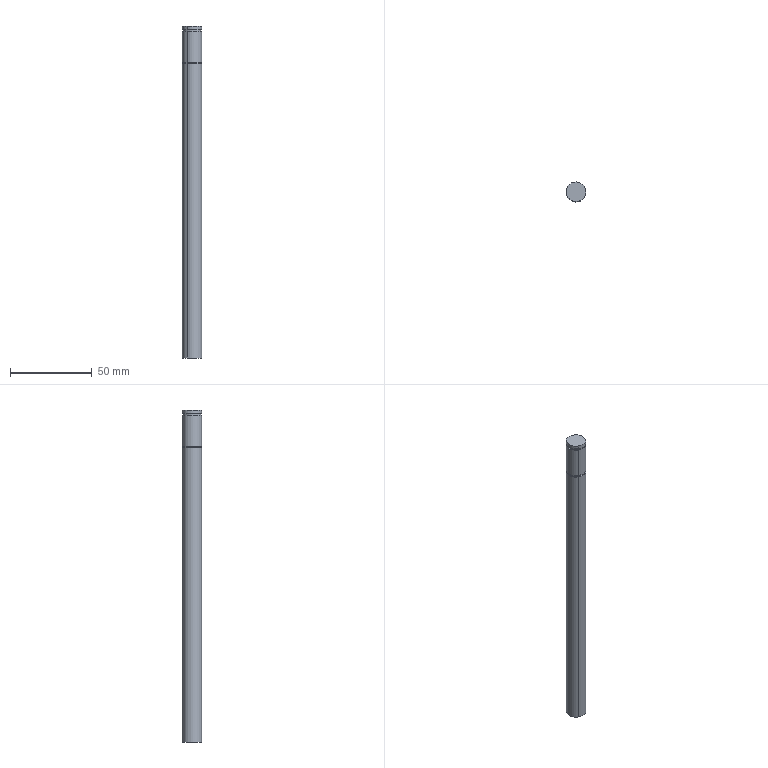Component | SolidWorks | TAR-02-026SmallPulleyAxis-1 | 1 solid | 16 faces | box 12 x 12 x 203 mm | volume 22911 mm3 | cylinder 10 | plane 6 | commonest cylinder face diameters 12 x6 10.8 x4
build123d program:
from build123d import *

# Parameters (mm, degrees)
SKETCH1_R           = 6
BOSS_EXTRUDE1_DEPTH = 2
SKETCH2_R           = 5.4
BOSS_EXTRUDE2_DEPTH = 1.1
SKETCH3_R           = 6
BOSS_EXTRUDE3_DEPTH = 19
SKETCH4_R           = 5.4
BOSS_EXTRUDE4_DEPTH = 1.1
SKETCH5_R           = 6
BOSS_EXTRUDE5_DEPTH = 179.8


with BuildPart() as part:
    # Sketch1 → Boss-Extrude1 (new body)
    with BuildSketch(Plane.XY):
        Circle(SKETCH1_R)
    extrude(amount=BOSS_EXTRUDE1_DEPTH)

    # Sketch2 → Boss-Extrude2 (add)
    with BuildSketch(Plane.XY.offset(2)):
        Circle(SKETCH2_R)
    extrude(amount=BOSS_EXTRUDE2_DEPTH)

    # Sketch3 → Boss-Extrude3 (add)
    with BuildSketch(Plane.XY.offset(3.1)):
        Circle(SKETCH3_R)
    extrude(amount=BOSS_EXTRUDE3_DEPTH)

    # Sketch4 → Boss-Extrude4 (add)
    with BuildSketch(Plane.XY.offset(22.1)):
        Circle(SKETCH4_R)
    extrude(amount=BOSS_EXTRUDE4_DEPTH)

    # Sketch5 → Boss-Extrude5 (add)
    with BuildSketch(Plane.XY.offset(23.2)):
        Circle(SKETCH5_R)
    extrude(amount=BOSS_EXTRUDE5_DEPTH)


solid = part.part

# Placed as in the assembly
solid = solid.moved(Location((-115.391, 9.288, 12.6), (180, 0, 0)))
STEP:
#1=COLOUR_RGB('',0.7922,0.8196,0.9333);
#2=FILL_AREA_STYLE_COLOUR('',#1);
#3=FILL_AREA_STYLE('',(#2));
#4=SURFACE_STYLE_FILL_AREA(#3);
#5=SURFACE_SIDE_STYLE('',(#4));
#6=SURFACE_STYLE_USAGE(.BOTH.,#5);
#7=PRESENTATION_STYLE_ASSIGNMENT((#6));
#8=CARTESIAN_POINT('',(-4.431,0.5734,-7.496));
#9=VERTEX_POINT('',#8);
#10=CARTESIAN_POINT('',(-4.655,0.1579,-7.496));
#11=VERTEX_POINT('',#10);
#12=CARTESIAN_POINT('',(-4.543,0.3657,-7.496));
#13=DIRECTION('',(0.,0.,-1.));
#14=DIRECTION('',(0.4758,0.8795,0.));
#15=AXIS2_PLACEMENT_3D('',#12,#13,#14);
#16=CIRCLE('',#15,0.2362);
#17=EDGE_CURVE('',#9,#11,#16,.T.);
#18=ORIENTED_EDGE('',*,*,#17,.F.);
#19=CARTESIAN_POINT('',(-4.431,0.5734,-0.4173));
#20=VERTEX_POINT('',#19);
#21=CARTESIAN_POINT('',(-4.431,0.5734,-7.496));
#22=DIRECTION('',(0.,0.,1.));
#23=VECTOR('',#22,39.37);
#24=LINE('',#21,#23);
#25=EDGE_CURVE('',#9,#20,#24,.T.);
#26=ORIENTED_EDGE('',*,*,#25,.T.);
#27=CARTESIAN_POINT('',(-4.655,0.1579,-0.4173));
#28=VERTEX_POINT('',#27);
#29=CARTESIAN_POINT('',(-4.543,0.3657,-0.4173));
#30=DIRECTION('',(0.,0.,-1.));
#31=DIRECTION('',(0.4758,0.8795,0.));
#32=AXIS2_PLACEMENT_3D('',#29,#30,#31);
#33=CIRCLE('',#32,0.2362);
#34=EDGE_CURVE('',#20,#28,#33,.T.);
#35=ORIENTED_EDGE('',*,*,#34,.T.);
#36=CARTESIAN_POINT('',(-4.655,0.1579,-7.496));
#37=DIRECTION('',(0.,0.,1.));
#38=VECTOR('',#37,39.37);
#39=LINE('',#36,#38);
#40=EDGE_CURVE('',#11,#28,#39,.T.);
#41=ORIENTED_EDGE('',*,*,#40,.F.);
#42=EDGE_LOOP('',(#18,#26,#35,#41));
#43=FACE_OUTER_BOUND('',#42,.T.);
#44=CARTESIAN_POINT('',(-4.543,0.3657,-7.496));
#45=DIRECTION('',(0.,0.,1.));
#46=DIRECTION('',(-0.4758,-0.8795,0.));
#47=AXIS2_PLACEMENT_3D('',#44,#45,#46);
#48=CYLINDRICAL_SURFACE('',#47,0.2362);
#49=ADVANCED_FACE('',(#43),#48,.T.);
#50=CARTESIAN_POINT('',(-4.442,0.5526,-0.4173));
#51=VERTEX_POINT('',#50);
#52=CARTESIAN_POINT('',(-4.644,0.1787,-0.4173));
#53=VERTEX_POINT('',#52);
#54=CARTESIAN_POINT('',(-4.543,0.3657,-0.4173));
#55=DIRECTION('',(0.,0.,-1.));
#56=DIRECTION('',(0.4758,0.8795,0.));
#57=AXIS2_PLACEMENT_3D('',#54,#55,#56);
#58=CIRCLE('',#57,0.2126);
#59=EDGE_CURVE('',#51,#53,#58,.T.);
#60=ORIENTED_EDGE('',*,*,#59,.F.);
#61=CARTESIAN_POINT('',(-4.442,0.5526,-0.374));
#62=VERTEX_POINT('',#61);
#63=CARTESIAN_POINT('',(-4.442,0.5526,-0.4173));
#64=DIRECTION('',(0.,0.,1.));
#65=VECTOR('',#64,39.37);
#66=LINE('',#63,#65);
#67=EDGE_CURVE('',#51,#62,#66,.T.);
#68=ORIENTED_EDGE('',*,*,#67,.T.);
#69=CARTESIAN_POINT('',(-4.644,0.1787,-0.374));
#70=VERTEX_POINT('',#69);
#71=CARTESIAN_POINT('',(-4.543,0.3657,-0.374));
#72=DIRECTION('',(0.,0.,-1.));
#73=DIRECTION('',(0.4758,0.8795,0.));
#74=AXIS2_PLACEMENT_3D('',#71,#72,#73);
#75=CIRCLE('',#74,0.2126);
#76=EDGE_CURVE('',#62,#70,#75,.T.);
#77=ORIENTED_EDGE('',*,*,#76,.T.);
#78=CARTESIAN_POINT('',(-4.644,0.1787,-0.4173));
#79=DIRECTION('',(0.,0.,1.));
#80=VECTOR('',#79,39.37);
#81=LINE('',#78,#80);
#82=EDGE_CURVE('',#53,#70,#81,.T.);
#83=ORIENTED_EDGE('',*,*,#82,.F.);
#84=EDGE_LOOP('',(#60,#68,#77,#83));
#85=FACE_OUTER_BOUND('',#84,.T.);
#86=CARTESIAN_POINT('',(-4.543,0.3657,-0.4173));
#87=DIRECTION('',(0.,0.,1.));
#88=DIRECTION('',(-0.4758,-0.8795,0.));
#89=AXIS2_PLACEMENT_3D('',#86,#87,#88);
#90=CYLINDRICAL_SURFACE('',#89,0.2126);
#91=ADVANCED_FACE('',(#85),#90,.T.);
#92=CARTESIAN_POINT('',(-4.431,0.5734,-0.374));
#93=VERTEX_POINT('',#92);
#94=CARTESIAN_POINT('',(-4.655,0.1579,-0.374));
#95=VERTEX_POINT('',#94);
#96=CARTESIAN_POINT('',(-4.543,0.3657,-0.374));
#97=DIRECTION('',(0.,0.,-1.));
#98=DIRECTION('',(0.4758,0.8795,0.));
#99=AXIS2_PLACEMENT_3D('',#96,#97,#98);
#100=CIRCLE('',#99,0.2362);
#101=EDGE_CURVE('',#93,#95,#100,.T.);
#102=ORIENTED_EDGE('',*,*,#101,.F.);
#103=CARTESIAN_POINT('',(-4.431,0.5734,0.374));
#104=VERTEX_POINT('',#103);
#105=CARTESIAN_POINT('',(-4.431,0.5734,-0.374));
#106=DIRECTION('',(0.,0.,1.));
#107=VECTOR('',#106,39.37);
#108=LINE('',#105,#107);
#109=EDGE_CURVE('',#93,#104,#108,.T.);
#110=ORIENTED_EDGE('',*,*,#109,.T.);
#111=CARTESIAN_POINT('',(-4.655,0.1579,0.374));
#112=VERTEX_POINT('',#111);
#113=CARTESIAN_POINT('',(-4.543,0.3657,0.374));
#114=DIRECTION('',(0.,0.,-1.));
#115=DIRECTION('',(0.4758,0.8795,0.));
#116=AXIS2_PLACEMENT_3D('',#113,#114,#115);
#117=CIRCLE('',#116,0.2362);
#118=EDGE_CURVE('',#104,#112,#117,.T.);
#119=ORIENTED_EDGE('',*,*,#118,.T.);
#120=CARTESIAN_POINT('',(-4.655,0.1579,-0.374));
#121=DIRECTION('',(0.,0.,1.));
#122=VECTOR('',#121,39.37);
#123=LINE('',#120,#122);
#124=EDGE_CURVE('',#95,#112,#123,.T.);
#125=ORIENTED_EDGE('',*,*,#124,.F.);
#126=EDGE_LOOP('',(#102,#110,#119,#125));
#127=FACE_OUTER_BOUND('',#126,.T.);
#128=CARTESIAN_POINT('',(-4.543,0.3657,-0.374));
#129=DIRECTION('',(0.,0.,1.));
#130=DIRECTION('',(-0.4758,-0.8795,0.));
#131=AXIS2_PLACEMENT_3D('',#128,#129,#130);
#132=CYLINDRICAL_SURFACE('',#131,0.2362);
#133=ADVANCED_FACE('',(#127),#132,.T.);
#134=CARTESIAN_POINT('',(-4.442,0.5526,0.374));
#135=VERTEX_POINT('',#134);
#136=CARTESIAN_POINT('',(-4.644,0.1787,0.374));
#137=VERTEX_POINT('',#136);
#138=CARTESIAN_POINT('',(-4.543,0.3657,0.374));
#139=DIRECTION('',(0.,0.,-1.));
#140=DIRECTION('',(0.4758,0.8795,0.));
#141=AXIS2_PLACEMENT_3D('',#138,#139,#140);
#142=CIRCLE('',#141,0.2126);
#143=EDGE_CURVE('',#135,#137,#142,.T.);
#144=ORIENTED_EDGE('',*,*,#143,.F.);
#145=CARTESIAN_POINT('',(-4.442,0.5526,0.4173));
#146=VERTEX_POINT('',#145);
#147=CARTESIAN_POINT('',(-4.442,0.5526,0.374));
#148=DIRECTION('',(0.,0.,1.));
#149=VECTOR('',#148,39.37);
#150=LINE('',#147,#149);
#151=EDGE_CURVE('',#135,#146,#150,.T.);
#152=ORIENTED_EDGE('',*,*,#151,.T.);
#153=CARTESIAN_POINT('',(-4.644,0.1787,0.4173));
#154=VERTEX_POINT('',#153);
#155=CARTESIAN_POINT('',(-4.543,0.3657,0.4173));
#156=DIRECTION('',(0.,0.,-1.));
#157=DIRECTION('',(0.4758,0.8795,0.));
#158=AXIS2_PLACEMENT_3D('',#155,#156,#157);
#159=CIRCLE('',#158,0.2126);
#160=EDGE_CURVE('',#146,#154,#159,.T.);
#161=ORIENTED_EDGE('',*,*,#160,.T.);
#162=CARTESIAN_POINT('',(-4.644,0.1787,0.374));
#163=DIRECTION('',(0.,0.,1.));
#164=VECTOR('',#163,39.37);
#165=LINE('',#162,#164);
#166=EDGE_CURVE('',#137,#154,#165,.T.);
#167=ORIENTED_EDGE('',*,*,#166,.F.);
#168=EDGE_LOOP('',(#144,#152,#161,#167));
#169=FACE_OUTER_BOUND('',#168,.T.);
#170=CARTESIAN_POINT('',(-4.543,0.3657,0.374));
#171=DIRECTION('',(0.,0.,1.));
#172=DIRECTION('',(-0.4758,-0.8795,0.));
#173=AXIS2_PLACEMENT_3D('',#170,#171,#172);
#174=CYLINDRICAL_SURFACE('',#173,0.2126);
#175=ADVANCED_FACE('',(#169),#174,.T.);
#176=CARTESIAN_POINT('',(-4.431,0.5734,0.4173));
#177=VERTEX_POINT('',#176);
#178=CARTESIAN_POINT('',(-4.655,0.1579,0.4173));
#179=VERTEX_POINT('',#178);
#180=CARTESIAN_POINT('',(-4.543,0.3657,0.4173));
#181=DIRECTION('',(0.,0.,-1.));
#182=DIRECTION('',(0.4758,0.8795,0.));
#183=AXIS2_PLACEMENT_3D('',#180,#181,#182);
#184=CIRCLE('',#183,0.2362);
#185=EDGE_CURVE('',#177,#179,#184,.T.);
#186=ORIENTED_EDGE('',*,*,#185,.F.);
#187=CARTESIAN_POINT('',(-4.431,0.5734,0.4961));
#188=VERTEX_POINT('',#187);
#189=CARTESIAN_POINT('',(-4.431,0.5734,0.4173));
#190=DIRECTION('',(0.,0.,1.));
#191=VECTOR('',#190,39.37);
#192=LINE('',#189,#191);
#193=EDGE_CURVE('',#177,#188,#192,.T.);
#194=ORIENTED_EDGE('',*,*,#193,.T.);
#195=CARTESIAN_POINT('',(-4.655,0.1579,0.4961));
#196=VERTEX_POINT('',#195);
#197=CARTESIAN_POINT('',(-4.543,0.3657,0.4961));
#198=DIRECTION('',(0.,0.,-1.));
#199=DIRECTION('',(0.4758,0.8795,0.));
#200=AXIS2_PLACEMENT_3D('',#197,#198,#199);
#201=CIRCLE('',#200,0.2362);
#202=EDGE_CURVE('',#188,#196,#201,.T.);
#203=ORIENTED_EDGE('',*,*,#202,.T.);
#204=CARTESIAN_POINT('',(-4.655,0.1579,0.4173));
#205=DIRECTION('',(0.,0.,1.));
#206=VECTOR('',#205,39.37);
#207=LINE('',#204,#206);
#208=EDGE_CURVE('',#179,#196,#207,.T.);
#209=ORIENTED_EDGE('',*,*,#208,.F.);
#210=EDGE_LOOP('',(#186,#194,#203,#209));
#211=FACE_OUTER_BOUND('',#210,.T.);
#212=CARTESIAN_POINT('',(-4.543,0.3657,0.4173));
#213=DIRECTION('',(0.,0.,1.));
#214=DIRECTION('',(-0.4758,-0.8795,0.));
#215=AXIS2_PLACEMENT_3D('',#212,#213,#214);
#216=CYLINDRICAL_SURFACE('',#215,0.2362);
#217=ADVANCED_FACE('',(#211),#216,.T.);
#218=ORIENTED_EDGE('',*,*,#193,.F.);
#219=CARTESIAN_POINT('',(-4.543,0.3657,0.4173));
#220=DIRECTION('',(0.,0.,-1.));
#221=DIRECTION('',(0.4758,0.8795,0.));
#222=AXIS2_PLACEMENT_3D('',#219,#220,#221);
#223=CIRCLE('',#222,0.2362);
#224=EDGE_CURVE('',#179,#177,#223,.T.);
#225=ORIENTED_EDGE('',*,*,#224,.F.);
#226=ORIENTED_EDGE('',*,*,#208,.T.);
#227=CARTESIAN_POINT('',(-4.543,0.3657,0.4961));
#228=DIRECTION('',(0.,0.,-1.));
#229=DIRECTION('',(0.4758,0.8795,0.));
#230=AXIS2_PLACEMENT_3D('',#227,#228,#229);
#231=CIRCLE('',#230,0.2362);
#232=EDGE_CURVE('',#196,#188,#231,.T.);
#233=ORIENTED_EDGE('',*,*,#232,.T.);
#234=EDGE_LOOP('',(#218,#225,#226,#233));
#235=FACE_OUTER_BOUND('',#234,.T.);
#236=CARTESIAN_POINT('',(-4.543,0.3657,0.4173));
#237=DIRECTION('',(0.,0.,1.));
#238=DIRECTION('',(-0.4758,-0.8795,0.));
#239=AXIS2_PLACEMENT_3D('',#236,#237,#238);
#240=CYLINDRICAL_SURFACE('',#239,0.2362);
#241=ADVANCED_FACE('',(#235),#240,.T.);
#242=CARTESIAN_POINT('',(-4.543,0.3657,0.4173));
#243=DIRECTION('',(0.,0.,-1.));
#244=DIRECTION('',(0.4758,0.8795,0.));
#245=AXIS2_PLACEMENT_3D('',#242,#243,#244);
#246=CIRCLE('',#245,0.2126);
#247=EDGE_CURVE('',#154,#146,#246,.T.);
#248=ORIENTED_EDGE('',*,*,#247,.F.);
#249=ORIENTED_EDGE('',*,*,#160,.F.);
#250=EDGE_LOOP('',(#248,#249));
#251=FACE_BOUND('',#250,.T.);
#252=ORIENTED_EDGE('',*,*,#224,.T.);
#253=ORIENTED_EDGE('',*,*,#185,.T.);
#254=EDGE_LOOP('',(#252,#253));
#255=FACE_OUTER_BOUND('',#254,.T.);
#256=CARTESIAN_POINT('',(-4.543,0.3657,0.4173));
#257=DIRECTION('',(0.,0.,-1.));
#258=DIRECTION('',(0.4758,0.8795,0.));
#259=AXIS2_PLACEMENT_3D('',#256,#257,#258);
#260=PLANE('',#259);
#261=ADVANCED_FACE('',(#251,#255),#260,.T.);
#262=ORIENTED_EDGE('',*,*,#232,.F.);
#263=ORIENTED_EDGE('',*,*,#202,.F.);
#264=EDGE_LOOP('',(#262,#263));
#265=FACE_OUTER_BOUND('',#264,.T.);
#266=CARTESIAN_POINT('',(-4.543,0.3657,0.4961));
#267=DIRECTION('',(0.,0.,-1.));
#268=DIRECTION('',(0.4758,0.8795,0.));
#269=AXIS2_PLACEMENT_3D('',#266,#267,#268);
#270=PLANE('',#269);
#271=ADVANCED_FACE('',(#265),#270,.F.);
#272=ORIENTED_EDGE('',*,*,#151,.F.);
#273=CARTESIAN_POINT('',(-4.543,0.3657,0.374));
#274=DIRECTION('',(0.,0.,-1.));
#275=DIRECTION('',(0.4758,0.8795,0.));
#276=AXIS2_PLACEMENT_3D('',#273,#274,#275);
#277=CIRCLE('',#276,0.2126);
#278=EDGE_CURVE('',#137,#135,#277,.T.);
#279=ORIENTED_EDGE('',*,*,#278,.F.);
#280=ORIENTED_EDGE('',*,*,#166,.T.);
#281=ORIENTED_EDGE('',*,*,#247,.T.);
#282=EDGE_LOOP('',(#272,#279,#280,#281));
#283=FACE_OUTER_BOUND('',#282,.T.);
#284=CARTESIAN_POINT('',(-4.543,0.3657,0.374));
#285=DIRECTION('',(0.,0.,1.));
#286=DIRECTION('',(-0.4758,-0.8795,0.));
#287=AXIS2_PLACEMENT_3D('',#284,#285,#286);
#288=CYLINDRICAL_SURFACE('',#287,0.2126);
#289=ADVANCED_FACE('',(#283),#288,.T.);
#290=ORIENTED_EDGE('',*,*,#109,.F.);
#291=CARTESIAN_POINT('',(-4.543,0.3657,-0.374));
#292=DIRECTION('',(0.,0.,-1.));
#293=DIRECTION('',(0.4758,0.8795,0.));
#294=AXIS2_PLACEMENT_3D('',#291,#292,#293);
#295=CIRCLE('',#294,0.2362);
#296=EDGE_CURVE('',#95,#93,#295,.T.);
#297=ORIENTED_EDGE('',*,*,#296,.F.);
#298=ORIENTED_EDGE('',*,*,#124,.T.);
#299=CARTESIAN_POINT('',(-4.543,0.3657,0.374));
#300=DIRECTION('',(0.,0.,-1.));
#301=DIRECTION('',(0.4758,0.8795,0.));
#302=AXIS2_PLACEMENT_3D('',#299,#300,#301);
#303=CIRCLE('',#302,0.2362);
#304=EDGE_CURVE('',#112,#104,#303,.T.);
#305=ORIENTED_EDGE('',*,*,#304,.T.);
#306=EDGE_LOOP('',(#290,#297,#298,#305));
#307=FACE_OUTER_BOUND('',#306,.T.);
#308=CARTESIAN_POINT('',(-4.543,0.3657,-0.374));
#309=DIRECTION('',(0.,0.,1.));
#310=DIRECTION('',(-0.4758,-0.8795,0.));
#311=AXIS2_PLACEMENT_3D('',#308,#309,#310);
#312=CYLINDRICAL_SURFACE('',#311,0.2362);
#313=ADVANCED_FACE('',(#307),#312,.T.);
#314=CARTESIAN_POINT('',(-4.543,0.3657,-0.374));
#315=DIRECTION('',(0.,0.,-1.));
#316=DIRECTION('',(0.4758,0.8795,0.));
#317=AXIS2_PLACEMENT_3D('',#314,#315,#316);
#318=CIRCLE('',#317,0.2126);
#319=EDGE_CURVE('',#70,#62,#318,.T.);
#320=ORIENTED_EDGE('',*,*,#319,.F.);
#321=ORIENTED_EDGE('',*,*,#76,.F.);
#322=EDGE_LOOP('',(#320,#321));
#323=FACE_BOUND('',#322,.T.);
#324=ORIENTED_EDGE('',*,*,#296,.T.);
#325=ORIENTED_EDGE('',*,*,#101,.T.);
#326=EDGE_LOOP('',(#324,#325));
#327=FACE_OUTER_BOUND('',#326,.T.);
#328=CARTESIAN_POINT('',(-4.543,0.3657,-0.374));
#329=DIRECTION('',(0.,0.,-1.));
#330=DIRECTION('',(0.4758,0.8795,0.));
#331=AXIS2_PLACEMENT_3D('',#328,#329,#330);
#332=PLANE('',#331);
#333=ADVANCED_FACE('',(#323,#327),#332,.T.);
#334=ORIENTED_EDGE('',*,*,#278,.T.);
#335=ORIENTED_EDGE('',*,*,#143,.T.);
#336=EDGE_LOOP('',(#334,#335));
#337=FACE_BOUND('',#336,.T.);
#338=ORIENTED_EDGE('',*,*,#304,.F.);
#339=ORIENTED_EDGE('',*,*,#118,.F.);
#340=EDGE_LOOP('',(#338,#339));
#341=FACE_OUTER_BOUND('',#340,.T.);
#342=CARTESIAN_POINT('',(-4.543,0.3657,0.374));
#343=DIRECTION('',(0.,0.,-1.));
#344=DIRECTION('',(0.4758,0.8795,0.));
#345=AXIS2_PLACEMENT_3D('',#342,#343,#344);
#346=PLANE('',#345);
#347=ADVANCED_FACE('',(#337,#341),#346,.F.);
#348=ORIENTED_EDGE('',*,*,#67,.F.);
#349=CARTESIAN_POINT('',(-4.543,0.3657,-0.4173));
#350=DIRECTION('',(0.,0.,-1.));
#351=DIRECTION('',(0.4758,0.8795,0.));
#352=AXIS2_PLACEMENT_3D('',#349,#350,#351);
#353=CIRCLE('',#352,0.2126);
#354=EDGE_CURVE('',#53,#51,#353,.T.);
#355=ORIENTED_EDGE('',*,*,#354,.F.);
#356=ORIENTED_EDGE('',*,*,#82,.T.);
#357=ORIENTED_EDGE('',*,*,#319,.T.);
#358=EDGE_LOOP('',(#348,#355,#356,#357));
#359=FACE_OUTER_BOUND('',#358,.T.);
#360=CARTESIAN_POINT('',(-4.543,0.3657,-0.4173));
#361=DIRECTION('',(0.,0.,1.));
#362=DIRECTION('',(-0.4758,-0.8795,0.));
#363=AXIS2_PLACEMENT_3D('',#360,#361,#362);
#364=CYLINDRICAL_SURFACE('',#363,0.2126);
#365=ADVANCED_FACE('',(#359),#364,.T.);
#366=ORIENTED_EDGE('',*,*,#25,.F.);
#367=CARTESIAN_POINT('',(-4.543,0.3657,-7.496));
#368=DIRECTION('',(0.,0.,-1.));
#369=DIRECTION('',(0.4758,0.8795,0.));
#370=AXIS2_PLACEMENT_3D('',#367,#368,#369);
#371=CIRCLE('',#370,0.2362);
#372=EDGE_CURVE('',#11,#9,#371,.T.);
#373=ORIENTED_EDGE('',*,*,#372,.F.);
#374=ORIENTED_EDGE('',*,*,#40,.T.);
#375=CARTESIAN_POINT('',(-4.543,0.3657,-0.4173));
#376=DIRECTION('',(0.,0.,-1.));
#377=DIRECTION('',(0.4758,0.8795,0.));
#378=AXIS2_PLACEMENT_3D('',#375,#376,#377);
#379=CIRCLE('',#378,0.2362);
#380=EDGE_CURVE('',#28,#20,#379,.T.);
#381=ORIENTED_EDGE('',*,*,#380,.T.);
#382=EDGE_LOOP('',(#366,#373,#374,#381));
#383=FACE_OUTER_BOUND('',#382,.T.);
#384=CARTESIAN_POINT('',(-4.543,0.3657,-7.496));
#385=DIRECTION('',(0.,0.,1.));
#386=DIRECTION('',(-0.4758,-0.8795,0.));
#387=AXIS2_PLACEMENT_3D('',#384,#385,#386);
#388=CYLINDRICAL_SURFACE('',#387,0.2362);
#389=ADVANCED_FACE('',(#383),#388,.T.);
#390=ORIENTED_EDGE('',*,*,#372,.T.);
#391=ORIENTED_EDGE('',*,*,#17,.T.);
#392=EDGE_LOOP('',(#390,#391));
#393=FACE_OUTER_BOUND('',#392,.T.);
#394=CARTESIAN_POINT('',(-4.543,0.3657,-7.496));
#395=DIRECTION('',(0.,0.,-1.));
#396=DIRECTION('',(0.4758,0.8795,0.));
#397=AXIS2_PLACEMENT_3D('',#394,#395,#396);
#398=PLANE('',#397);
#399=ADVANCED_FACE('',(#393),#398,.T.);
#400=ORIENTED_EDGE('',*,*,#354,.T.);
#401=ORIENTED_EDGE('',*,*,#59,.T.);
#402=EDGE_LOOP('',(#400,#401));
#403=FACE_BOUND('',#402,.T.);
#404=ORIENTED_EDGE('',*,*,#380,.F.);
#405=ORIENTED_EDGE('',*,*,#34,.F.);
#406=EDGE_LOOP('',(#404,#405));
#407=FACE_OUTER_BOUND('',#406,.T.);
#408=CARTESIAN_POINT('',(-4.543,0.3657,-0.4173));
#409=DIRECTION('',(0.,0.,-1.));
#410=DIRECTION('',(0.4758,0.8795,0.));
#411=AXIS2_PLACEMENT_3D('',#408,#409,#410);
#412=PLANE('',#411);
#413=ADVANCED_FACE('',(#403,#407),#412,.F.);
#414=CLOSED_SHELL('',(#49,#91,#133,#175,#217,#241,#261,#271,#289,#313,#333,#347,#365,#389,#399,#413));
#415=MANIFOLD_SOLID_BREP('',#414);
#416=STYLED_ITEM('',(#7),#415);
#417=(LENGTH_UNIT()NAMED_UNIT(*)SI_UNIT($,.METRE.));
#418=LENGTH_MEASURE_WITH_UNIT(LENGTH_MEASURE(0.0254),#417);
#419=DIMENSIONAL_EXPONENTS(1.,0.,0.,0.,0.,0.,0.);
#420=(CONVERSION_BASED_UNIT('',#418)LENGTH_UNIT()NAMED_UNIT(#419));
#421=UNCERTAINTY_MEASURE_WITH_UNIT(LENGTH_MEASURE(0.00001),#420,'','');
#422=(NAMED_UNIT(*)PLANE_ANGLE_UNIT()SI_UNIT($,.RADIAN.));
#423=(NAMED_UNIT(*)SI_UNIT($,.STERADIAN.)SOLID_ANGLE_UNIT());
#424=(GEOMETRIC_REPRESENTATION_CONTEXT(3)GLOBAL_UNCERTAINTY_ASSIGNED_CONTEXT((#421))GLOBAL_UNIT_ASSIGNED_CONTEXT((#420,#422,#423))REPRESENTATION_CONTEXT('',''));
#425=MECHANICAL_DESIGN_GEOMETRIC_PRESENTATION_REPRESENTATION('',(#416),#424);
#426=CARTESIAN_POINT('',(0.,0.,0.));
#427=DIRECTION('',(0.,0.,1.));
#428=DIRECTION('',(1.,0.,0.));
#429=AXIS2_PLACEMENT_3D('',#426,#427,#428);
#430=(LENGTH_UNIT()NAMED_UNIT(*)SI_UNIT($,.METRE.));
#431=LENGTH_MEASURE_WITH_UNIT(LENGTH_MEASURE(0.0254),#430);
#432=DIMENSIONAL_EXPONENTS(1.,0.,0.,0.,0.,0.,0.);
#433=(CONVERSION_BASED_UNIT('',#431)LENGTH_UNIT()NAMED_UNIT(#432));
#434=UNCERTAINTY_MEASURE_WITH_UNIT(LENGTH_MEASURE(0.00001),#433,'','');
#435=(NAMED_UNIT(*)PLANE_ANGLE_UNIT()SI_UNIT($,.RADIAN.));
#436=(NAMED_UNIT(*)SI_UNIT($,.STERADIAN.)SOLID_ANGLE_UNIT());
#437=(GEOMETRIC_REPRESENTATION_CONTEXT(3)GLOBAL_UNCERTAINTY_ASSIGNED_CONTEXT((#434))GLOBAL_UNIT_ASSIGNED_CONTEXT((#433,#435,#436))REPRESENTATION_CONTEXT('',''));
#438=ADVANCED_BREP_SHAPE_REPRESENTATION('',(#415,#429),#437);
#439=PRESENTATION_LAYER_ASSIGNMENT('','',(#416));